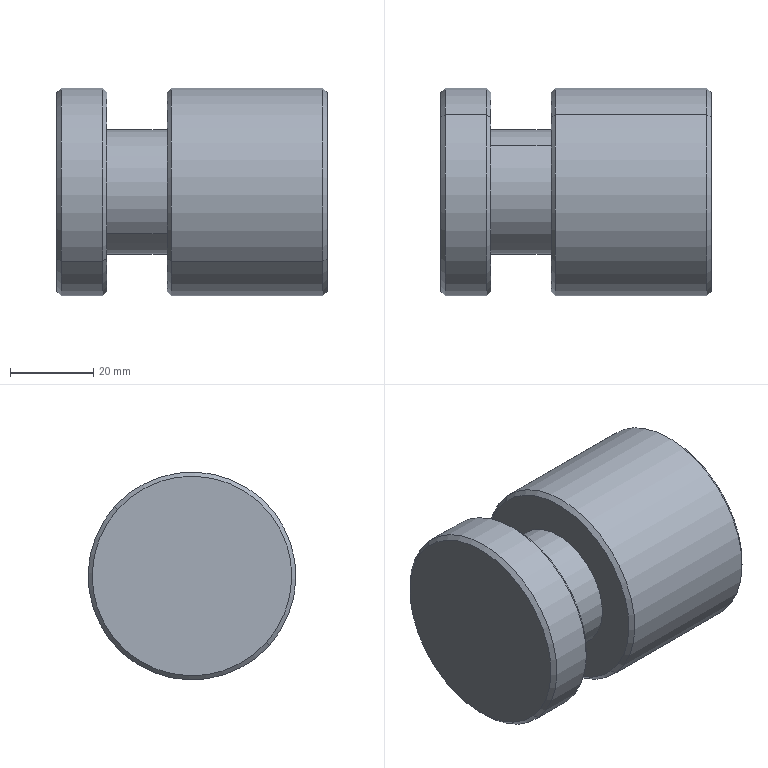Component | SolidWorks | ZN-A-009-1 | 1 solid | 22 faces | box 65 x 50 x 50 mm | volume 92410 mm3 | cone 10 | cylinder 8 | plane 4 | commonest cylinder face diameters 50 x4 30 x2 20.5 x2
build123d program:
from build123d import *

# Parameters (mm, degrees)
SKETCH2_R                  = 25
BOSS_EXTRUDE1_DEPTH        = 32.5
M22X1_5_TAPPED_HOLE1_D     = 20.5
M22X1_5_TAPPED_HOLE1_DEPTH = 48.5
M22X1_5_TAPPED_HOLE1_TIP   = 6.159
SKETCH5_W                  = 18.324
SKETCH5_H                  = 14.5
CHAMFER1_SIZE              = 1


with BuildPart() as part:
    # Sketch2 → Boss-Extrude1 (new, symmetric)
    with BuildSketch(Plane(origin=(0, 0, 0), x_dir=(1, 0, 0), z_dir=(0, 1, 0))):
        with Locations(Location((0, 0, 0), (0, 0, 270))):
            Circle(SKETCH2_R)
    extrude(amount=BOSS_EXTRUDE1_DEPTH, both=True)

    # M22x1.5 Tapped Hole1
    with Locations(Plane(origin=(0, -32.5, 0), x_dir=(-1, 0, 0), z_dir=(0, -1, 0))):
        with Locations((0, 0)):
            Hole(M22X1_5_TAPPED_HOLE1_D / 2, depth=M22X1_5_TAPPED_HOLE1_DEPTH)
            with Locations((0, 0, -(M22X1_5_TAPPED_HOLE1_DEPTH + M22X1_5_TAPPED_HOLE1_TIP / 2))):  # 118° drill point
                Cone(0, M22X1_5_TAPPED_HOLE1_D / 2, M22X1_5_TAPPED_HOLE1_TIP, mode=Mode.SUBTRACT)

    # Sketch5 → Cut-Revolve1 (revolve, cut)
    with BuildSketch(Plane.XY, mode=Mode.PRIVATE) as cut_revolve1_sk:
        with Locations((24.162, 13.25)):
            Rectangle(SKETCH5_W, SKETCH5_H)
    revolve(cut_revolve1_sk.sketch.rotate(Axis((0, 32.5, 0), (0, -1, 0)), 270), axis=Axis((0, 32.5, 0), (0, -1, 0)), mode=Mode.SUBTRACT)

    # Chamfer1
    chamfer1_edges = [part.edges().sort_by_distance(p)[0] for p in [
        (0, 6, -25),
        (0, 20.5, -25),
        (0, -32.5, -25),
        (0, 32.5, -25),
    ]]
    chamfer(chamfer1_edges, length=CHAMFER1_SIZE)


solid = part.part

# Placed as in the assembly
solid = solid.moved(Location((571.892, 232.499, 100), (0, 0, 90)))
STEP:
#1=CARTESIAN_POINT('',(21.236,9.857,4.568));
#2=VERTEX_POINT('',#1);
#3=CARTESIAN_POINT('',(21.236,8.45,3.306));
#4=VERTEX_POINT('',#3);
#5=CARTESIAN_POINT('',(21.236,9.154,3.937));
#6=DIRECTION('',(-1.,0.,-0.));
#7=DIRECTION('',(0.,0.7446,0.6675));
#8=AXIS2_PLACEMENT_3D('',#5,#6,#7);
#9=CIRCLE('',#8,0.9449);
#10=EDGE_CURVE('',#2,#4,#9,.T.);
#11=ORIENTED_EDGE('',*,*,#10,.F.);
#12=CARTESIAN_POINT('',(21.275,9.886,4.594));
#13=VERTEX_POINT('',#12);
#14=CARTESIAN_POINT('',(21.236,9.857,4.568));
#15=DIRECTION('',(0.7071,0.5265,0.472));
#16=VECTOR('',#15,39.37);
#17=LINE('',#14,#16);
#18=EDGE_CURVE('',#2,#13,#17,.T.);
#19=ORIENTED_EDGE('',*,*,#18,.T.);
#20=CARTESIAN_POINT('',(21.275,8.421,3.28));
#21=VERTEX_POINT('',#20);
#22=CARTESIAN_POINT('',(21.275,9.154,3.937));
#23=DIRECTION('',(1.,-0.,0.));
#24=DIRECTION('',(0.,0.7446,0.6675));
#25=AXIS2_PLACEMENT_3D('',#22,#23,#24);
#26=CIRCLE('',#25,0.9843);
#27=EDGE_CURVE('',#21,#13,#26,.T.);
#28=ORIENTED_EDGE('',*,*,#27,.F.);
#29=CARTESIAN_POINT('',(21.236,8.45,3.306));
#30=DIRECTION('',(0.7071,-0.5265,-0.472));
#31=VECTOR('',#30,39.37);
#32=LINE('',#29,#31);
#33=EDGE_CURVE('',#4,#21,#32,.T.);
#34=ORIENTED_EDGE('',*,*,#33,.F.);
#35=EDGE_LOOP('',(#11,#19,#28,#34));
#36=FACE_OUTER_BOUND('',#35,.T.);
#37=CARTESIAN_POINT('',(21.236,9.154,3.937));
#38=DIRECTION('',(1.,-0.,0.));
#39=DIRECTION('',(0.,-0.7446,-0.6675));
#40=AXIS2_PLACEMENT_3D('',#37,#38,#39);
#41=CONICAL_SURFACE('',#40,0.9449,0.7854);
#42=ADVANCED_FACE('',(#36),#41,.T.);
#43=CARTESIAN_POINT('',(23.795,8.45,3.306));
#44=VERTEX_POINT('',#43);
#45=CARTESIAN_POINT('',(23.795,9.857,4.568));
#46=VERTEX_POINT('',#45);
#47=CARTESIAN_POINT('',(23.795,9.154,3.937));
#48=DIRECTION('',(1.,-0.,0.));
#49=DIRECTION('',(0.,0.7446,0.6675));
#50=AXIS2_PLACEMENT_3D('',#47,#48,#49);
#51=CIRCLE('',#50,0.9449);
#52=EDGE_CURVE('',#44,#46,#51,.T.);
#53=ORIENTED_EDGE('',*,*,#52,.F.);
#54=CARTESIAN_POINT('',(23.756,8.421,3.28));
#55=VERTEX_POINT('',#54);
#56=CARTESIAN_POINT('',(23.756,8.421,3.28));
#57=DIRECTION('',(-0.7071,-0.5265,-0.472));
#58=VECTOR('',#57,39.37);
#59=LINE('',#56,#58);
#60=EDGE_CURVE('',#44,#55,#59,.T.);
#61=ORIENTED_EDGE('',*,*,#60,.T.);
#62=CARTESIAN_POINT('',(23.756,9.886,4.594));
#63=VERTEX_POINT('',#62);
#64=CARTESIAN_POINT('',(23.756,9.154,3.937));
#65=DIRECTION('',(-1.,0.,-0.));
#66=DIRECTION('',(0.,0.7446,0.6675));
#67=AXIS2_PLACEMENT_3D('',#64,#65,#66);
#68=CIRCLE('',#67,0.9843);
#69=EDGE_CURVE('',#63,#55,#68,.T.);
#70=ORIENTED_EDGE('',*,*,#69,.F.);
#71=CARTESIAN_POINT('',(23.756,9.886,4.594));
#72=DIRECTION('',(-0.7071,0.5265,0.472));
#73=VECTOR('',#72,39.37);
#74=LINE('',#71,#73);
#75=EDGE_CURVE('',#46,#63,#74,.T.);
#76=ORIENTED_EDGE('',*,*,#75,.F.);
#77=EDGE_LOOP('',(#53,#61,#70,#76));
#78=FACE_OUTER_BOUND('',#77,.T.);
#79=CARTESIAN_POINT('',(23.756,9.154,3.937));
#80=DIRECTION('',(-1.,0.,-0.));
#81=DIRECTION('',(0.,0.7446,0.6675));
#82=AXIS2_PLACEMENT_3D('',#79,#80,#81);
#83=CONICAL_SURFACE('',#82,0.9843,0.7854);
#84=ADVANCED_FACE('',(#78),#83,.T.);
#85=CARTESIAN_POINT('',(21.708,8.45,3.306));
#86=VERTEX_POINT('',#85);
#87=CARTESIAN_POINT('',(21.708,9.857,4.568));
#88=VERTEX_POINT('',#87);
#89=CARTESIAN_POINT('',(21.708,9.154,3.937));
#90=DIRECTION('',(1.,-0.,0.));
#91=DIRECTION('',(0.,-0.7446,-0.6675));
#92=AXIS2_PLACEMENT_3D('',#89,#90,#91);
#93=CIRCLE('',#92,0.9449);
#94=EDGE_CURVE('',#86,#88,#93,.T.);
#95=ORIENTED_EDGE('',*,*,#94,.F.);
#96=CARTESIAN_POINT('',(21.669,8.421,3.28));
#97=VERTEX_POINT('',#96);
#98=CARTESIAN_POINT('',(21.708,8.45,3.306));
#99=DIRECTION('',(-0.7071,-0.5265,-0.472));
#100=VECTOR('',#99,39.37);
#101=LINE('',#98,#100);
#102=EDGE_CURVE('',#86,#97,#101,.T.);
#103=ORIENTED_EDGE('',*,*,#102,.T.);
#104=CARTESIAN_POINT('',(21.669,9.886,4.594));
#105=VERTEX_POINT('',#104);
#106=CARTESIAN_POINT('',(21.669,9.154,3.937));
#107=DIRECTION('',(-1.,0.,-0.));
#108=DIRECTION('',(0.,-0.7446,-0.6675));
#109=AXIS2_PLACEMENT_3D('',#106,#107,#108);
#110=CIRCLE('',#109,0.9843);
#111=EDGE_CURVE('',#105,#97,#110,.T.);
#112=ORIENTED_EDGE('',*,*,#111,.F.);
#113=CARTESIAN_POINT('',(21.708,9.857,4.568));
#114=DIRECTION('',(-0.7071,0.5265,0.472));
#115=VECTOR('',#114,39.37);
#116=LINE('',#113,#115);
#117=EDGE_CURVE('',#88,#105,#116,.T.);
#118=ORIENTED_EDGE('',*,*,#117,.F.);
#119=EDGE_LOOP('',(#95,#103,#112,#118));
#120=FACE_OUTER_BOUND('',#119,.T.);
#121=CARTESIAN_POINT('',(21.708,9.154,3.937));
#122=DIRECTION('',(-1.,0.,-0.));
#123=DIRECTION('',(0.,0.7446,0.6675));
#124=AXIS2_PLACEMENT_3D('',#121,#122,#123);
#125=CONICAL_SURFACE('',#124,0.9449,0.7854);
#126=ADVANCED_FACE('',(#120),#125,.T.);
#127=CARTESIAN_POINT('',(22.279,9.857,4.568));
#128=VERTEX_POINT('',#127);
#129=CARTESIAN_POINT('',(22.279,8.45,3.306));
#130=VERTEX_POINT('',#129);
#131=CARTESIAN_POINT('',(22.279,9.154,3.937));
#132=DIRECTION('',(-1.,0.,-0.));
#133=DIRECTION('',(0.,0.7446,0.6675));
#134=AXIS2_PLACEMENT_3D('',#131,#132,#133);
#135=CIRCLE('',#134,0.9449);
#136=EDGE_CURVE('',#128,#130,#135,.T.);
#137=ORIENTED_EDGE('',*,*,#136,.F.);
#138=CARTESIAN_POINT('',(22.319,9.886,4.594));
#139=VERTEX_POINT('',#138);
#140=CARTESIAN_POINT('',(22.279,9.857,4.568));
#141=DIRECTION('',(0.7071,0.5265,0.472));
#142=VECTOR('',#141,39.37);
#143=LINE('',#140,#142);
#144=EDGE_CURVE('',#128,#139,#143,.T.);
#145=ORIENTED_EDGE('',*,*,#144,.T.);
#146=CARTESIAN_POINT('',(22.319,8.421,3.28));
#147=VERTEX_POINT('',#146);
#148=CARTESIAN_POINT('',(22.319,9.154,3.937));
#149=DIRECTION('',(1.,-0.,0.));
#150=DIRECTION('',(0.,0.7446,0.6675));
#151=AXIS2_PLACEMENT_3D('',#148,#149,#150);
#152=CIRCLE('',#151,0.9843);
#153=EDGE_CURVE('',#147,#139,#152,.T.);
#154=ORIENTED_EDGE('',*,*,#153,.F.);
#155=CARTESIAN_POINT('',(22.279,8.45,3.306));
#156=DIRECTION('',(0.7071,-0.5265,-0.472));
#157=VECTOR('',#156,39.37);
#158=LINE('',#155,#157);
#159=EDGE_CURVE('',#130,#147,#158,.T.);
#160=ORIENTED_EDGE('',*,*,#159,.F.);
#161=EDGE_LOOP('',(#137,#145,#154,#160));
#162=FACE_OUTER_BOUND('',#161,.T.);
#163=CARTESIAN_POINT('',(22.279,9.154,3.937));
#164=DIRECTION('',(1.,-0.,0.));
#165=DIRECTION('',(0.,-0.7446,-0.6675));
#166=AXIS2_PLACEMENT_3D('',#163,#164,#165);
#167=CONICAL_SURFACE('',#166,0.9449,0.7854);
#168=ADVANCED_FACE('',(#162),#167,.T.);
#169=ORIENTED_EDGE('',*,*,#27,.T.);
#170=CARTESIAN_POINT('',(21.236,9.886,4.594));
#171=DIRECTION('',(1.,-0.,0.));
#172=VECTOR('',#171,39.37);
#173=LINE('',#170,#172);
#174=EDGE_CURVE('',#13,#105,#173,.T.);
#175=ORIENTED_EDGE('',*,*,#174,.T.);
#176=ORIENTED_EDGE('',*,*,#111,.T.);
#177=CARTESIAN_POINT('',(21.236,8.421,3.28));
#178=DIRECTION('',(1.,-0.,0.));
#179=VECTOR('',#178,39.37);
#180=LINE('',#177,#179);
#181=EDGE_CURVE('',#21,#97,#180,.T.);
#182=ORIENTED_EDGE('',*,*,#181,.F.);
#183=EDGE_LOOP('',(#169,#175,#176,#182));
#184=FACE_OUTER_BOUND('',#183,.T.);
#185=CARTESIAN_POINT('',(21.236,9.154,3.937));
#186=DIRECTION('',(1.,-0.,0.));
#187=DIRECTION('',(0.,-0.7446,-0.6675));
#188=AXIS2_PLACEMENT_3D('',#185,#186,#187);
#189=CYLINDRICAL_SURFACE('',#188,0.9843);
#190=ADVANCED_FACE('',(#184),#189,.T.);
#191=CARTESIAN_POINT('',(22.279,9.593,4.331));
#192=VERTEX_POINT('',#191);
#193=CARTESIAN_POINT('',(22.279,8.714,3.543));
#194=VERTEX_POINT('',#193);
#195=CARTESIAN_POINT('',(22.279,9.154,3.937));
#196=DIRECTION('',(-1.,0.,-0.));
#197=DIRECTION('',(0.,0.7446,0.6675));
#198=AXIS2_PLACEMENT_3D('',#195,#196,#197);
#199=CIRCLE('',#198,0.5906);
#200=EDGE_CURVE('',#192,#194,#199,.T.);
#201=ORIENTED_EDGE('',*,*,#200,.T.);
#202=CARTESIAN_POINT('',(21.708,8.714,3.543));
#203=VERTEX_POINT('',#202);
#204=CARTESIAN_POINT('',(21.236,8.714,3.543));
#205=DIRECTION('',(-1.,0.,-0.));
#206=VECTOR('',#205,39.37);
#207=LINE('',#204,#206);
#208=EDGE_CURVE('',#194,#203,#207,.T.);
#209=ORIENTED_EDGE('',*,*,#208,.T.);
#210=CARTESIAN_POINT('',(21.708,9.593,4.331));
#211=VERTEX_POINT('',#210);
#212=CARTESIAN_POINT('',(21.708,9.154,3.937));
#213=DIRECTION('',(-1.,0.,-0.));
#214=DIRECTION('',(0.,0.7446,0.6675));
#215=AXIS2_PLACEMENT_3D('',#212,#213,#214);
#216=CIRCLE('',#215,0.5906);
#217=EDGE_CURVE('',#211,#203,#216,.T.);
#218=ORIENTED_EDGE('',*,*,#217,.F.);
#219=CARTESIAN_POINT('',(21.236,9.593,4.331));
#220=DIRECTION('',(-1.,0.,-0.));
#221=VECTOR('',#220,39.37);
#222=LINE('',#219,#221);
#223=EDGE_CURVE('',#192,#211,#222,.T.);
#224=ORIENTED_EDGE('',*,*,#223,.F.);
#225=EDGE_LOOP('',(#201,#209,#218,#224));
#226=FACE_OUTER_BOUND('',#225,.T.);
#227=CARTESIAN_POINT('',(21.236,9.154,3.937));
#228=DIRECTION('',(-1.,0.,-0.));
#229=DIRECTION('',(0.,0.7446,0.6675));
#230=AXIS2_PLACEMENT_3D('',#227,#228,#229);
#231=CYLINDRICAL_SURFACE('',#230,0.5906);
#232=ADVANCED_FACE('',(#226),#231,.T.);
#233=CARTESIAN_POINT('',(21.886,9.454,4.206));
#234=VERTEX_POINT('',#233);
#235=CARTESIAN_POINT('',(21.886,8.853,3.668));
#236=VERTEX_POINT('',#235);
#237=CARTESIAN_POINT('',(21.886,9.154,3.937));
#238=DIRECTION('',(1.,-0.,0.));
#239=DIRECTION('',(0.,-0.7446,-0.6675));
#240=AXIS2_PLACEMENT_3D('',#237,#238,#239);
#241=CIRCLE('',#240,0.4035);
#242=EDGE_CURVE('',#234,#236,#241,.T.);
#243=ORIENTED_EDGE('',*,*,#242,.F.);
#244=CARTESIAN_POINT('',(23.795,9.454,4.206));
#245=VERTEX_POINT('',#244);
#246=CARTESIAN_POINT('',(23.795,9.454,4.206));
#247=DIRECTION('',(1.,-0.,0.));
#248=VECTOR('',#247,39.37);
#249=LINE('',#246,#248);
#250=EDGE_CURVE('',#234,#245,#249,.T.);
#251=ORIENTED_EDGE('',*,*,#250,.T.);
#252=CARTESIAN_POINT('',(23.795,8.853,3.668));
#253=VERTEX_POINT('',#252);
#254=CARTESIAN_POINT('',(23.795,9.154,3.937));
#255=DIRECTION('',(1.,-0.,0.));
#256=DIRECTION('',(0.,-0.7446,-0.6675));
#257=AXIS2_PLACEMENT_3D('',#254,#255,#256);
#258=CIRCLE('',#257,0.4035);
#259=EDGE_CURVE('',#245,#253,#258,.T.);
#260=ORIENTED_EDGE('',*,*,#259,.T.);
#261=CARTESIAN_POINT('',(23.795,8.853,3.668));
#262=DIRECTION('',(1.,-0.,0.));
#263=VECTOR('',#262,39.37);
#264=LINE('',#261,#263);
#265=EDGE_CURVE('',#236,#253,#264,.T.);
#266=ORIENTED_EDGE('',*,*,#265,.F.);
#267=EDGE_LOOP('',(#243,#251,#260,#266));
#268=FACE_OUTER_BOUND('',#267,.T.);
#269=CARTESIAN_POINT('',(23.795,9.154,3.937));
#270=DIRECTION('',(1.,-0.,0.));
#271=DIRECTION('',(0.,-0.7446,-0.6675));
#272=AXIS2_PLACEMENT_3D('',#269,#270,#271);
#273=CYLINDRICAL_SURFACE('',#272,0.4035);
#274=ADVANCED_FACE('',(#268),#273,.F.);
#275=CARTESIAN_POINT('',(21.643,9.154,3.937));
#276=VERTEX_POINT('',#275);
#277=CARTESIAN_POINT('',(21.886,8.853,3.668));
#278=DIRECTION('',(0.515,-0.6383,-0.5721));
#279=VECTOR('',#278,39.37);
#280=LINE('',#277,#279);
#281=EDGE_CURVE('',#276,#236,#280,.T.);
#282=ORIENTED_EDGE('',*,*,#281,.F.);
#283=CARTESIAN_POINT('',(21.886,9.454,4.206));
#284=DIRECTION('',(0.515,0.6383,0.5721));
#285=VECTOR('',#284,39.37);
#286=LINE('',#283,#285);
#287=EDGE_CURVE('',#276,#234,#286,.T.);
#288=ORIENTED_EDGE('',*,*,#287,.T.);
#289=ORIENTED_EDGE('',*,*,#242,.T.);
#290=EDGE_LOOP('',(#282,#288,#289));
#291=FACE_OUTER_BOUND('',#290,.T.);
#292=CARTESIAN_POINT('',(21.886,9.154,3.937));
#293=DIRECTION('',(1.,-0.,0.));
#294=DIRECTION('',(0.,-0.7446,-0.6675));
#295=AXIS2_PLACEMENT_3D('',#292,#293,#294);
#296=CONICAL_SURFACE('',#295,0.4035,1.03);
#297=ADVANCED_FACE('',(#291),#296,.F.);
#298=ORIENTED_EDGE('',*,*,#153,.T.);
#299=CARTESIAN_POINT('',(21.236,9.886,4.594));
#300=DIRECTION('',(1.,-0.,0.));
#301=VECTOR('',#300,39.37);
#302=LINE('',#299,#301);
#303=EDGE_CURVE('',#139,#63,#302,.T.);
#304=ORIENTED_EDGE('',*,*,#303,.T.);
#305=ORIENTED_EDGE('',*,*,#69,.T.);
#306=CARTESIAN_POINT('',(21.236,8.421,3.28));
#307=DIRECTION('',(1.,-0.,0.));
#308=VECTOR('',#307,39.37);
#309=LINE('',#306,#308);
#310=EDGE_CURVE('',#147,#55,#309,.T.);
#311=ORIENTED_EDGE('',*,*,#310,.F.);
#312=EDGE_LOOP('',(#298,#304,#305,#311));
#313=FACE_OUTER_BOUND('',#312,.T.);
#314=CARTESIAN_POINT('',(21.236,9.154,3.937));
#315=DIRECTION('',(1.,-0.,0.));
#316=DIRECTION('',(0.,-0.7446,-0.6675));
#317=AXIS2_PLACEMENT_3D('',#314,#315,#316);
#318=CYLINDRICAL_SURFACE('',#317,0.9843);
#319=ADVANCED_FACE('',(#313),#318,.T.);
#320=ORIENTED_EDGE('',*,*,#303,.F.);
#321=CARTESIAN_POINT('',(22.319,9.154,3.937));
#322=DIRECTION('',(1.,-0.,0.));
#323=DIRECTION('',(0.,0.7446,0.6675));
#324=AXIS2_PLACEMENT_3D('',#321,#322,#323);
#325=CIRCLE('',#324,0.9843);
#326=EDGE_CURVE('',#139,#147,#325,.T.);
#327=ORIENTED_EDGE('',*,*,#326,.T.);
#328=ORIENTED_EDGE('',*,*,#310,.T.);
#329=CARTESIAN_POINT('',(23.756,9.154,3.937));
#330=DIRECTION('',(-1.,0.,-0.));
#331=DIRECTION('',(0.,0.7446,0.6675));
#332=AXIS2_PLACEMENT_3D('',#329,#330,#331);
#333=CIRCLE('',#332,0.9843);
#334=EDGE_CURVE('',#55,#63,#333,.T.);
#335=ORIENTED_EDGE('',*,*,#334,.T.);
#336=EDGE_LOOP('',(#320,#327,#328,#335));
#337=FACE_OUTER_BOUND('',#336,.T.);
#338=CARTESIAN_POINT('',(21.236,9.154,3.937));
#339=DIRECTION('',(1.,-0.,0.));
#340=DIRECTION('',(0.,-0.7446,-0.6675));
#341=AXIS2_PLACEMENT_3D('',#338,#339,#340);
#342=CYLINDRICAL_SURFACE('',#341,0.9843);
#343=ADVANCED_FACE('',(#337),#342,.T.);
#344=CARTESIAN_POINT('',(23.795,9.154,3.937));
#345=DIRECTION('',(1.,-0.,0.));
#346=DIRECTION('',(0.,0.7446,0.6675));
#347=AXIS2_PLACEMENT_3D('',#344,#345,#346);
#348=CIRCLE('',#347,0.9449);
#349=EDGE_CURVE('',#46,#44,#348,.T.);
#350=ORIENTED_EDGE('',*,*,#349,.T.);
#351=ORIENTED_EDGE('',*,*,#52,.T.);
#352=EDGE_LOOP('',(#350,#351));
#353=FACE_OUTER_BOUND('',#352,.T.);
#354=CARTESIAN_POINT('',(23.795,9.154,3.937));
#355=DIRECTION('',(1.,-0.,0.));
#356=DIRECTION('',(0.,-0.7446,-0.6675));
#357=AXIS2_PLACEMENT_3D('',#354,#355,#356);
#358=CIRCLE('',#357,0.4035);
#359=EDGE_CURVE('',#253,#245,#358,.T.);
#360=ORIENTED_EDGE('',*,*,#359,.F.);
#361=ORIENTED_EDGE('',*,*,#259,.F.);
#362=EDGE_LOOP('',(#360,#361));
#363=FACE_BOUND('',#362,.T.);
#364=CARTESIAN_POINT('',(23.795,9.154,3.937));
#365=DIRECTION('',(-1.,0.,-0.));
#366=DIRECTION('',(0.,0.7446,0.6675));
#367=AXIS2_PLACEMENT_3D('',#364,#365,#366);
#368=PLANE('',#367);
#369=ADVANCED_FACE('',(#353,#363),#368,.F.);
#370=ORIENTED_EDGE('',*,*,#287,.F.);
#371=ORIENTED_EDGE('',*,*,#281,.T.);
#372=CARTESIAN_POINT('',(21.886,9.154,3.937));
#373=DIRECTION('',(1.,-0.,0.));
#374=DIRECTION('',(0.,-0.7446,-0.6675));
#375=AXIS2_PLACEMENT_3D('',#372,#373,#374);
#376=CIRCLE('',#375,0.4035);
#377=EDGE_CURVE('',#236,#234,#376,.T.);
#378=ORIENTED_EDGE('',*,*,#377,.T.);
#379=EDGE_LOOP('',(#370,#371,#378));
#380=FACE_OUTER_BOUND('',#379,.T.);
#381=CARTESIAN_POINT('',(21.886,9.154,3.937));
#382=DIRECTION('',(1.,-0.,0.));
#383=DIRECTION('',(0.,-0.7446,-0.6675));
#384=AXIS2_PLACEMENT_3D('',#381,#382,#383);
#385=CONICAL_SURFACE('',#384,0.4035,1.03);
#386=ADVANCED_FACE('',(#380),#385,.F.);
#387=ORIENTED_EDGE('',*,*,#250,.F.);
#388=ORIENTED_EDGE('',*,*,#377,.F.);
#389=ORIENTED_EDGE('',*,*,#265,.T.);
#390=ORIENTED_EDGE('',*,*,#359,.T.);
#391=EDGE_LOOP('',(#387,#388,#389,#390));
#392=FACE_OUTER_BOUND('',#391,.T.);
#393=CARTESIAN_POINT('',(23.795,9.154,3.937));
#394=DIRECTION('',(1.,-0.,0.));
#395=DIRECTION('',(0.,-0.7446,-0.6675));
#396=AXIS2_PLACEMENT_3D('',#393,#394,#395);
#397=CYLINDRICAL_SURFACE('',#396,0.4035);
#398=ADVANCED_FACE('',(#392),#397,.F.);
#399=CARTESIAN_POINT('',(22.279,9.154,3.937));
#400=DIRECTION('',(-1.,0.,-0.));
#401=DIRECTION('',(0.,0.7446,0.6675));
#402=AXIS2_PLACEMENT_3D('',#399,#400,#401);
#403=CIRCLE('',#402,0.9449);
#404=EDGE_CURVE('',#130,#128,#403,.T.);
#405=ORIENTED_EDGE('',*,*,#404,.T.);
#406=ORIENTED_EDGE('',*,*,#136,.T.);
#407=EDGE_LOOP('',(#405,#406));
#408=FACE_OUTER_BOUND('',#407,.T.);
#409=ORIENTED_EDGE('',*,*,#200,.F.);
#410=CARTESIAN_POINT('',(22.279,9.154,3.937));
#411=DIRECTION('',(-1.,0.,-0.));
#412=DIRECTION('',(0.,0.7446,0.6675));
#413=AXIS2_PLACEMENT_3D('',#410,#411,#412);
#414=CIRCLE('',#413,0.5906);
#415=EDGE_CURVE('',#194,#192,#414,.T.);
#416=ORIENTED_EDGE('',*,*,#415,.F.);
#417=EDGE_LOOP('',(#409,#416));
#418=FACE_BOUND('',#417,.T.);
#419=CARTESIAN_POINT('',(22.279,9.548,3.497));
#420=DIRECTION('',(-1.,0.,-0.));
#421=DIRECTION('',(0.,0.7446,0.6675));
#422=AXIS2_PLACEMENT_3D('',#419,#420,#421);
#423=PLANE('',#422);
#424=ADVANCED_FACE('',(#408,#418),#423,.T.);
#425=CARTESIAN_POINT('',(21.708,9.154,3.937));
#426=DIRECTION('',(1.,-0.,0.));
#427=DIRECTION('',(0.,-0.7446,-0.6675));
#428=AXIS2_PLACEMENT_3D('',#425,#426,#427);
#429=CIRCLE('',#428,0.9449);
#430=EDGE_CURVE('',#88,#86,#429,.T.);
#431=ORIENTED_EDGE('',*,*,#430,.T.);
#432=ORIENTED_EDGE('',*,*,#94,.T.);
#433=EDGE_LOOP('',(#431,#432));
#434=FACE_OUTER_BOUND('',#433,.T.);
#435=ORIENTED_EDGE('',*,*,#217,.T.);
#436=CARTESIAN_POINT('',(21.708,9.154,3.937));
#437=DIRECTION('',(-1.,0.,-0.));
#438=DIRECTION('',(0.,0.7446,0.6675));
#439=AXIS2_PLACEMENT_3D('',#436,#437,#438);
#440=CIRCLE('',#439,0.5906);
#441=EDGE_CURVE('',#203,#211,#440,.T.);
#442=ORIENTED_EDGE('',*,*,#441,.T.);
#443=EDGE_LOOP('',(#435,#442));
#444=FACE_BOUND('',#443,.T.);
#445=CARTESIAN_POINT('',(21.708,9.548,3.497));
#446=DIRECTION('',(1.,-0.,0.));
#447=DIRECTION('',(-0.,-0.7446,-0.6675));
#448=AXIS2_PLACEMENT_3D('',#445,#446,#447);
#449=PLANE('',#448);
#450=ADVANCED_FACE('',(#434,#444),#449,.T.);
#451=ORIENTED_EDGE('',*,*,#208,.F.);
#452=ORIENTED_EDGE('',*,*,#415,.T.);
#453=ORIENTED_EDGE('',*,*,#223,.T.);
#454=ORIENTED_EDGE('',*,*,#441,.F.);
#455=EDGE_LOOP('',(#451,#452,#453,#454));
#456=FACE_OUTER_BOUND('',#455,.T.);
#457=CARTESIAN_POINT('',(21.236,9.154,3.937));
#458=DIRECTION('',(-1.,0.,-0.));
#459=DIRECTION('',(0.,0.7446,0.6675));
#460=AXIS2_PLACEMENT_3D('',#457,#458,#459);
#461=CYLINDRICAL_SURFACE('',#460,0.5906);
#462=ADVANCED_FACE('',(#456),#461,.T.);
#463=CARTESIAN_POINT('',(21.236,9.154,3.937));
#464=DIRECTION('',(-1.,0.,-0.));
#465=DIRECTION('',(0.,0.7446,0.6675));
#466=AXIS2_PLACEMENT_3D('',#463,#464,#465);
#467=CIRCLE('',#466,0.9449);
#468=EDGE_CURVE('',#4,#2,#467,.T.);
#469=ORIENTED_EDGE('',*,*,#468,.T.);
#470=ORIENTED_EDGE('',*,*,#10,.T.);
#471=EDGE_LOOP('',(#469,#470));
#472=FACE_OUTER_BOUND('',#471,.T.);
#473=CARTESIAN_POINT('',(21.236,9.154,3.937));
#474=DIRECTION('',(-1.,0.,-0.));
#475=DIRECTION('',(0.,0.7446,0.6675));
#476=AXIS2_PLACEMENT_3D('',#473,#474,#475);
#477=PLANE('',#476);
#478=ADVANCED_FACE('',(#472),#477,.T.);
#479=ORIENTED_EDGE('',*,*,#174,.F.);
#480=CARTESIAN_POINT('',(21.275,9.154,3.937));
#481=DIRECTION('',(1.,-0.,0.));
#482=DIRECTION('',(0.,0.7446,0.6675));
#483=AXIS2_PLACEMENT_3D('',#480,#481,#482);
#484=CIRCLE('',#483,0.9843);
#485=EDGE_CURVE('',#13,#21,#484,.T.);
#486=ORIENTED_EDGE('',*,*,#485,.T.);
#487=ORIENTED_EDGE('',*,*,#181,.T.);
#488=CARTESIAN_POINT('',(21.669,9.154,3.937));
#489=DIRECTION('',(-1.,0.,-0.));
#490=DIRECTION('',(0.,-0.7446,-0.6675));
#491=AXIS2_PLACEMENT_3D('',#488,#489,#490);
#492=CIRCLE('',#491,0.9843);
#493=EDGE_CURVE('',#97,#105,#492,.T.);
#494=ORIENTED_EDGE('',*,*,#493,.T.);
#495=EDGE_LOOP('',(#479,#486,#487,#494));
#496=FACE_OUTER_BOUND('',#495,.T.);
#497=CARTESIAN_POINT('',(21.236,9.154,3.937));
#498=DIRECTION('',(1.,-0.,0.));
#499=DIRECTION('',(0.,-0.7446,-0.6675));
#500=AXIS2_PLACEMENT_3D('',#497,#498,#499);
#501=CYLINDRICAL_SURFACE('',#500,0.9843);
#502=ADVANCED_FACE('',(#496),#501,.T.);
#503=ORIENTED_EDGE('',*,*,#144,.F.);
#504=ORIENTED_EDGE('',*,*,#404,.F.);
#505=ORIENTED_EDGE('',*,*,#159,.T.);
#506=ORIENTED_EDGE('',*,*,#326,.F.);
#507=EDGE_LOOP('',(#503,#504,#505,#506));
#508=FACE_OUTER_BOUND('',#507,.T.);
#509=CARTESIAN_POINT('',(22.279,9.154,3.937));
#510=DIRECTION('',(1.,-0.,0.));
#511=DIRECTION('',(0.,-0.7446,-0.6675));
#512=AXIS2_PLACEMENT_3D('',#509,#510,#511);
#513=CONICAL_SURFACE('',#512,0.9449,0.7854);
#514=ADVANCED_FACE('',(#508),#513,.T.);
#515=ORIENTED_EDGE('',*,*,#102,.F.);
#516=ORIENTED_EDGE('',*,*,#430,.F.);
#517=ORIENTED_EDGE('',*,*,#117,.T.);
#518=ORIENTED_EDGE('',*,*,#493,.F.);
#519=EDGE_LOOP('',(#515,#516,#517,#518));
#520=FACE_OUTER_BOUND('',#519,.T.);
#521=CARTESIAN_POINT('',(21.708,9.154,3.937));
#522=DIRECTION('',(-1.,0.,-0.));
#523=DIRECTION('',(0.,0.7446,0.6675));
#524=AXIS2_PLACEMENT_3D('',#521,#522,#523);
#525=CONICAL_SURFACE('',#524,0.9449,0.7854);
#526=ADVANCED_FACE('',(#520),#525,.T.);
#527=ORIENTED_EDGE('',*,*,#60,.F.);
#528=ORIENTED_EDGE('',*,*,#349,.F.);
#529=ORIENTED_EDGE('',*,*,#75,.T.);
#530=ORIENTED_EDGE('',*,*,#334,.F.);
#531=EDGE_LOOP('',(#527,#528,#529,#530));
#532=FACE_OUTER_BOUND('',#531,.T.);
#533=CARTESIAN_POINT('',(23.756,9.154,3.937));
#534=DIRECTION('',(-1.,0.,-0.));
#535=DIRECTION('',(0.,0.7446,0.6675));
#536=AXIS2_PLACEMENT_3D('',#533,#534,#535);
#537=CONICAL_SURFACE('',#536,0.9843,0.7854);
#538=ADVANCED_FACE('',(#532),#537,.T.);
#539=ORIENTED_EDGE('',*,*,#18,.F.);
#540=ORIENTED_EDGE('',*,*,#468,.F.);
#541=ORIENTED_EDGE('',*,*,#33,.T.);
#542=ORIENTED_EDGE('',*,*,#485,.F.);
#543=EDGE_LOOP('',(#539,#540,#541,#542));
#544=FACE_OUTER_BOUND('',#543,.T.);
#545=CARTESIAN_POINT('',(21.236,9.154,3.937));
#546=DIRECTION('',(1.,-0.,0.));
#547=DIRECTION('',(0.,-0.7446,-0.6675));
#548=AXIS2_PLACEMENT_3D('',#545,#546,#547);
#549=CONICAL_SURFACE('',#548,0.9449,0.7854);
#550=ADVANCED_FACE('',(#544),#549,.T.);
#551=CLOSED_SHELL('',(#42,#84,#126,#168,#190,#232,#274,#297,#319,#343,#369,#386,#398,#424,#450,#462,#478,#502,#514,#526,#538,#550));
#552=MANIFOLD_SOLID_BREP('',#551);
#553=CARTESIAN_POINT('',(0.,0.,0.));
#554=DIRECTION('',(0.,0.,1.));
#555=DIRECTION('',(1.,0.,0.));
#556=AXIS2_PLACEMENT_3D('',#553,#554,#555);
#557=(LENGTH_UNIT()NAMED_UNIT(*)SI_UNIT($,.METRE.));
#558=LENGTH_MEASURE_WITH_UNIT(LENGTH_MEASURE(0.0254),#557);
#559=DIMENSIONAL_EXPONENTS(1.,0.,0.,0.,0.,0.,0.);
#560=(CONVERSION_BASED_UNIT('',#558)LENGTH_UNIT()NAMED_UNIT(#559));
#561=UNCERTAINTY_MEASURE_WITH_UNIT(LENGTH_MEASURE(0.00001),#560,'','');
#562=(NAMED_UNIT(*)PLANE_ANGLE_UNIT()SI_UNIT($,.RADIAN.));
#563=(NAMED_UNIT(*)SI_UNIT($,.STERADIAN.)SOLID_ANGLE_UNIT());
#564=(GEOMETRIC_REPRESENTATION_CONTEXT(3)GLOBAL_UNCERTAINTY_ASSIGNED_CONTEXT((#561))GLOBAL_UNIT_ASSIGNED_CONTEXT((#560,#562,#563))REPRESENTATION_CONTEXT('',''));
#565=ADVANCED_BREP_SHAPE_REPRESENTATION('',(#552,#556),#564);
#566=COLOUR_RGB('',0.7922,0.8196,0.9333);
#567=FILL_AREA_STYLE_COLOUR('',#566);
#568=FILL_AREA_STYLE('',(#567));
#569=SURFACE_STYLE_FILL_AREA(#568);
#570=SURFACE_SIDE_STYLE('',(#569));
#571=SURFACE_STYLE_USAGE(.BOTH.,#570);
#572=PRESENTATION_STYLE_ASSIGNMENT((#571));
#573=STYLED_ITEM('',(#572),#552);
#574=(LENGTH_UNIT()NAMED_UNIT(*)SI_UNIT($,.METRE.));
#575=LENGTH_MEASURE_WITH_UNIT(LENGTH_MEASURE(0.0254),#574);
#576=DIMENSIONAL_EXPONENTS(1.,0.,0.,0.,0.,0.,0.);
#577=(CONVERSION_BASED_UNIT('',#575)LENGTH_UNIT()NAMED_UNIT(#576));
#578=UNCERTAINTY_MEASURE_WITH_UNIT(LENGTH_MEASURE(0.00001),#577,'','');
#579=(NAMED_UNIT(*)PLANE_ANGLE_UNIT()SI_UNIT($,.RADIAN.));
#580=(NAMED_UNIT(*)SI_UNIT($,.STERADIAN.)SOLID_ANGLE_UNIT());
#581=(GEOMETRIC_REPRESENTATION_CONTEXT(3)GLOBAL_UNCERTAINTY_ASSIGNED_CONTEXT((#578))GLOBAL_UNIT_ASSIGNED_CONTEXT((#577,#579,#580))REPRESENTATION_CONTEXT('',''));
#582=MECHANICAL_DESIGN_GEOMETRIC_PRESENTATION_REPRESENTATION('',(#573),#581);
#583=PRESENTATION_LAYER_ASSIGNMENT('','',(#573));